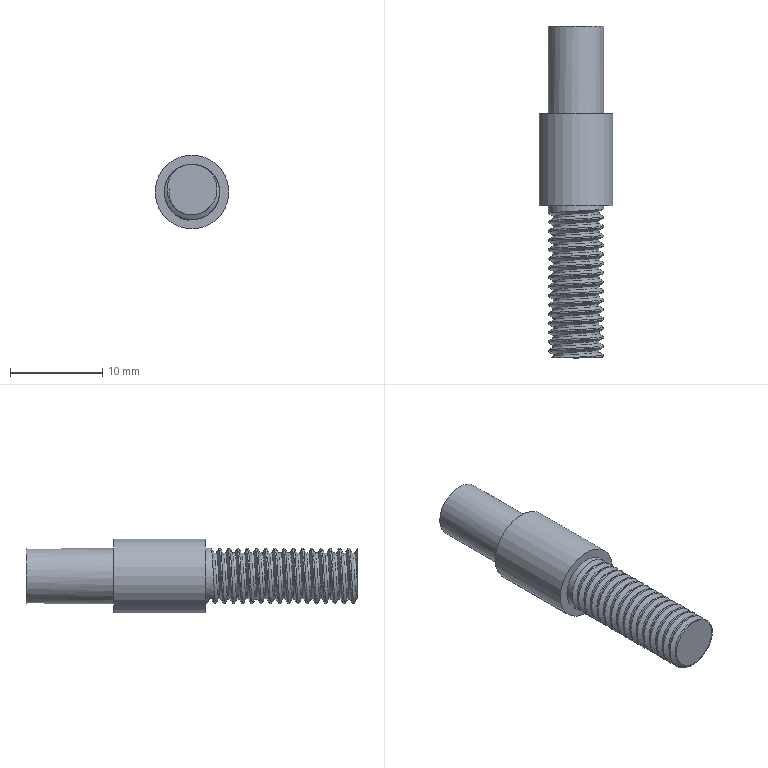Component | NX | STUD | 1 solid | 12 faces | volume 1143 mm3 | plane 5 | cylinder 4 | spline 3 | commonest cylinder face diameters 6 x2 8 x1 5 x1